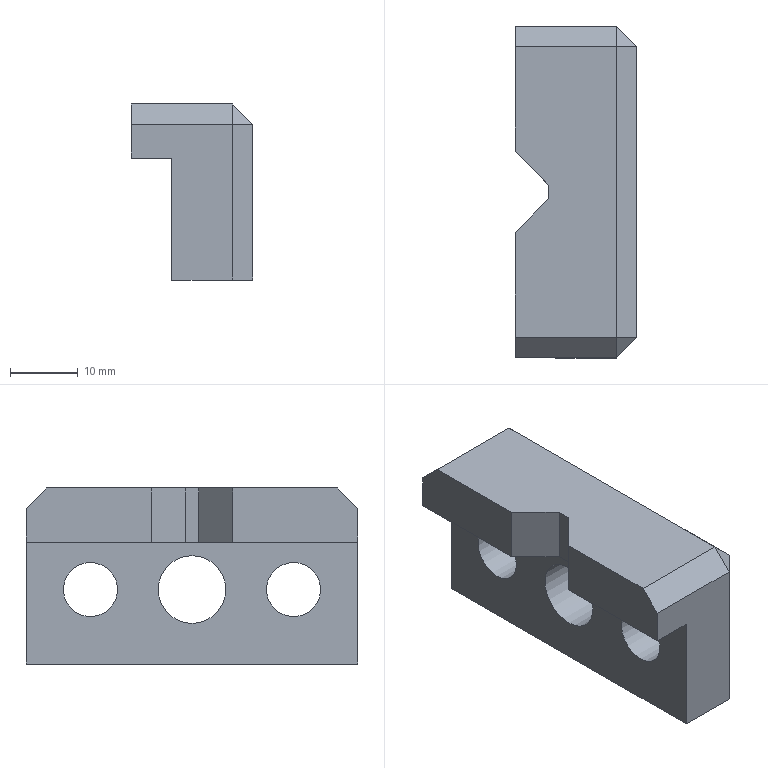Component | NX | MOVABLE_JAW | 1 solid | 22 faces | volume 14631 mm3 | plane 19 | cylinder 3 | commonest cylinder face diameters 8 x2 10 x1